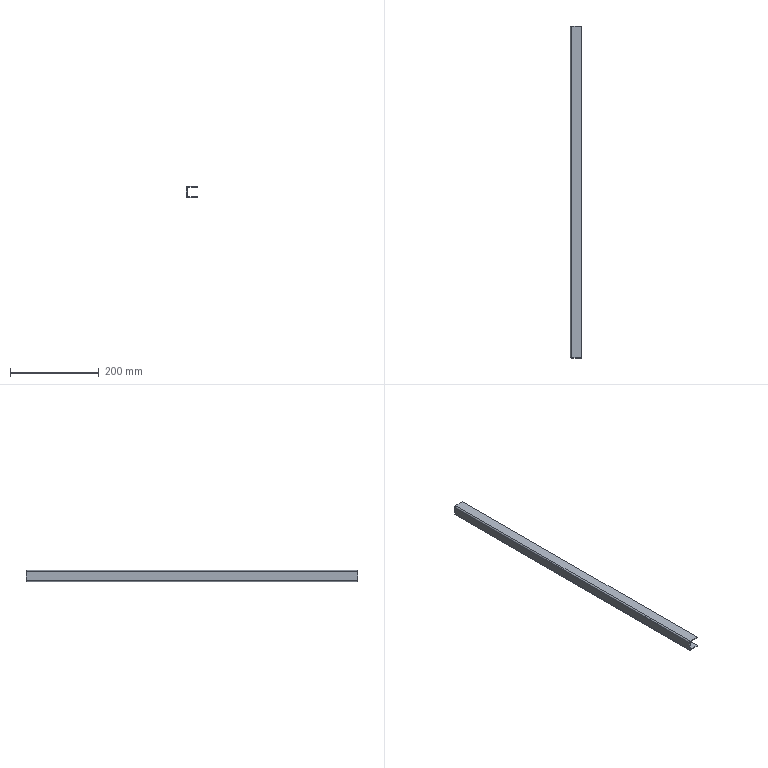Component | SolidWorks | Crossbeam.1(Item52)-1_Crossbeam.1(Item52)-1 | 1 solid | 22 faces | box 25 x 750 x 25 mm | volume 103925 mm3 | plane 18 | cylinder 4 | commonest cylinder face diameters 6 x2 2 x2 | material Plain Carbon Steel
STEP:
#1=CARTESIAN_POINT('',(-15.748,-14.764,-44.173));
#2=VERTEX_POINT('',#1);
#3=CARTESIAN_POINT('',(-15.669,-14.764,-44.173));
#4=VERTEX_POINT('',#3);
#5=CARTESIAN_POINT('',(-15.748,-14.764,-44.173));
#6=DIRECTION('',(1.,0.,-0.));
#7=VECTOR('',#6,39.37);
#8=LINE('',#5,#7);
#9=EDGE_CURVE('',#2,#4,#8,.T.);
#10=ORIENTED_EDGE('',*,*,#9,.F.);
#11=CARTESIAN_POINT('',(-15.63,-14.764,-44.291));
#12=VERTEX_POINT('',#11);
#13=CARTESIAN_POINT('',(-15.63,-14.764,-44.173));
#14=DIRECTION('',(-0.,1.,0.));
#15=DIRECTION('',(0.,0.,1.));
#16=AXIS2_PLACEMENT_3D('',#13,#14,#15);
#17=CIRCLE('',#16,0.1181);
#18=EDGE_CURVE('',#12,#2,#17,.T.);
#19=ORIENTED_EDGE('',*,*,#18,.F.);
#20=CARTESIAN_POINT('',(-15.63,-14.764,-44.213));
#21=VERTEX_POINT('',#20);
#22=CARTESIAN_POINT('',(-15.63,-14.764,-44.213));
#23=DIRECTION('',(-0.,0.,-1.));
#24=VECTOR('',#23,39.37);
#25=LINE('',#22,#24);
#26=EDGE_CURVE('',#21,#12,#25,.T.);
#27=ORIENTED_EDGE('',*,*,#26,.F.);
#28=CARTESIAN_POINT('',(-15.63,-14.764,-44.173));
#29=DIRECTION('',(-0.,1.,0.));
#30=DIRECTION('',(0.,0.,1.));
#31=AXIS2_PLACEMENT_3D('',#28,#29,#30);
#32=CIRCLE('',#31,0.03937);
#33=EDGE_CURVE('',#21,#4,#32,.T.);
#34=ORIENTED_EDGE('',*,*,#33,.T.);
#35=EDGE_LOOP('',(#10,#19,#27,#34));
#36=FACE_OUTER_BOUND('',#35,.T.);
#37=CARTESIAN_POINT('',(-15.748,-14.764,-44.173));
#38=DIRECTION('',(0.,-1.,-0.));
#39=DIRECTION('',(0.,-0.,1.));
#40=AXIS2_PLACEMENT_3D('',#37,#38,#39);
#41=PLANE('',#40);
#42=ADVANCED_FACE('',(#36),#41,.T.);
#43=CARTESIAN_POINT('',(-15.748,-14.764,-43.425));
#44=VERTEX_POINT('',#43);
#45=CARTESIAN_POINT('',(-15.748,-14.764,-44.291));
#46=DIRECTION('',(-0.,-0.,1.));
#47=VECTOR('',#46,39.37);
#48=LINE('',#45,#47);
#49=EDGE_CURVE('',#2,#44,#48,.T.);
#50=ORIENTED_EDGE('',*,*,#49,.F.);
#51=ORIENTED_EDGE('',*,*,#9,.T.);
#52=CARTESIAN_POINT('',(-15.669,-14.764,-43.425));
#53=VERTEX_POINT('',#52);
#54=CARTESIAN_POINT('',(-15.669,-14.764,-44.291));
#55=DIRECTION('',(-0.,-0.,1.));
#56=VECTOR('',#55,39.37);
#57=LINE('',#54,#56);
#58=EDGE_CURVE('',#4,#53,#57,.T.);
#59=ORIENTED_EDGE('',*,*,#58,.T.);
#60=CARTESIAN_POINT('',(-15.669,-14.764,-43.425));
#61=DIRECTION('',(-1.,-0.,0.));
#62=VECTOR('',#61,39.37);
#63=LINE('',#60,#62);
#64=EDGE_CURVE('',#53,#44,#63,.T.);
#65=ORIENTED_EDGE('',*,*,#64,.T.);
#66=EDGE_LOOP('',(#50,#51,#59,#65));
#67=FACE_OUTER_BOUND('',#66,.T.);
#68=CARTESIAN_POINT('',(-15.63,-14.764,-44.213));
#69=DIRECTION('',(0.,-1.,-0.));
#70=DIRECTION('',(0.,-0.,1.));
#71=AXIS2_PLACEMENT_3D('',#68,#69,#70);
#72=PLANE('',#71);
#73=ADVANCED_FACE('',(#67),#72,.T.);
#74=CARTESIAN_POINT('',(-15.63,14.764,-44.291));
#75=VERTEX_POINT('',#74);
#76=CARTESIAN_POINT('',(-15.63,14.764,-44.213));
#77=VERTEX_POINT('',#76);
#78=CARTESIAN_POINT('',(-15.63,14.764,-44.291));
#79=DIRECTION('',(0.,-0.,1.));
#80=VECTOR('',#79,39.37);
#81=LINE('',#78,#80);
#82=EDGE_CURVE('',#75,#77,#81,.T.);
#83=ORIENTED_EDGE('',*,*,#82,.F.);
#84=CARTESIAN_POINT('',(-15.748,14.764,-44.173));
#85=VERTEX_POINT('',#84);
#86=CARTESIAN_POINT('',(-15.63,14.764,-44.173));
#87=DIRECTION('',(-0.,1.,0.));
#88=DIRECTION('',(0.,0.,1.));
#89=AXIS2_PLACEMENT_3D('',#86,#87,#88);
#90=CIRCLE('',#89,0.1181);
#91=EDGE_CURVE('',#75,#85,#90,.T.);
#92=ORIENTED_EDGE('',*,*,#91,.T.);
#93=CARTESIAN_POINT('',(-15.669,14.764,-44.173));
#94=VERTEX_POINT('',#93);
#95=CARTESIAN_POINT('',(-15.669,14.764,-44.173));
#96=DIRECTION('',(-1.,-0.,0.));
#97=VECTOR('',#96,39.37);
#98=LINE('',#95,#97);
#99=EDGE_CURVE('',#94,#85,#98,.T.);
#100=ORIENTED_EDGE('',*,*,#99,.F.);
#101=CARTESIAN_POINT('',(-15.63,14.764,-44.173));
#102=DIRECTION('',(-0.,1.,0.));
#103=DIRECTION('',(0.,0.,1.));
#104=AXIS2_PLACEMENT_3D('',#101,#102,#103);
#105=CIRCLE('',#104,0.03937);
#106=EDGE_CURVE('',#77,#94,#105,.T.);
#107=ORIENTED_EDGE('',*,*,#106,.F.);
#108=EDGE_LOOP('',(#83,#92,#100,#107));
#109=FACE_OUTER_BOUND('',#108,.T.);
#110=CARTESIAN_POINT('',(-15.63,14.764,-44.291));
#111=DIRECTION('',(-0.,1.,0.));
#112=DIRECTION('',(-0.,0.,-1.));
#113=AXIS2_PLACEMENT_3D('',#110,#111,#112);
#114=PLANE('',#113);
#115=ADVANCED_FACE('',(#109),#114,.T.);
#116=CARTESIAN_POINT('',(-14.764,14.764,-44.291));
#117=VERTEX_POINT('',#116);
#118=CARTESIAN_POINT('',(-14.764,14.764,-44.291));
#119=DIRECTION('',(-1.,-0.,-0.));
#120=VECTOR('',#119,39.37);
#121=LINE('',#118,#120);
#122=EDGE_CURVE('',#117,#75,#121,.T.);
#123=ORIENTED_EDGE('',*,*,#122,.T.);
#124=ORIENTED_EDGE('',*,*,#82,.T.);
#125=CARTESIAN_POINT('',(-14.764,14.764,-44.213));
#126=VERTEX_POINT('',#125);
#127=CARTESIAN_POINT('',(-14.764,14.764,-44.213));
#128=DIRECTION('',(-1.,-0.,-0.));
#129=VECTOR('',#128,39.37);
#130=LINE('',#127,#129);
#131=EDGE_CURVE('',#126,#77,#130,.T.);
#132=ORIENTED_EDGE('',*,*,#131,.F.);
#133=CARTESIAN_POINT('',(-14.764,14.764,-44.213));
#134=DIRECTION('',(-0.,0.,-1.));
#135=VECTOR('',#134,39.37);
#136=LINE('',#133,#135);
#137=EDGE_CURVE('',#126,#117,#136,.T.);
#138=ORIENTED_EDGE('',*,*,#137,.T.);
#139=EDGE_LOOP('',(#123,#124,#132,#138));
#140=FACE_OUTER_BOUND('',#139,.T.);
#141=CARTESIAN_POINT('',(-15.669,14.764,-44.173));
#142=DIRECTION('',(-0.,1.,0.));
#143=DIRECTION('',(-0.,0.,-1.));
#144=AXIS2_PLACEMENT_3D('',#141,#142,#143);
#145=PLANE('',#144);
#146=ADVANCED_FACE('',(#140),#145,.T.);
#147=CARTESIAN_POINT('',(-15.63,-14.764,-43.307));
#148=VERTEX_POINT('',#147);
#149=CARTESIAN_POINT('',(-15.63,-14.764,-43.386));
#150=VERTEX_POINT('',#149);
#151=CARTESIAN_POINT('',(-15.63,-14.764,-43.307));
#152=DIRECTION('',(0.,0.,-1.));
#153=VECTOR('',#152,39.37);
#154=LINE('',#151,#153);
#155=EDGE_CURVE('',#148,#150,#154,.T.);
#156=ORIENTED_EDGE('',*,*,#155,.F.);
#157=CARTESIAN_POINT('',(-15.63,-14.764,-43.425));
#158=DIRECTION('',(-0.,1.,0.));
#159=DIRECTION('',(0.,0.,1.));
#160=AXIS2_PLACEMENT_3D('',#157,#158,#159);
#161=CIRCLE('',#160,0.1181);
#162=EDGE_CURVE('',#44,#148,#161,.T.);
#163=ORIENTED_EDGE('',*,*,#162,.F.);
#164=ORIENTED_EDGE('',*,*,#64,.F.);
#165=CARTESIAN_POINT('',(-15.63,-14.764,-43.425));
#166=DIRECTION('',(-0.,1.,0.));
#167=DIRECTION('',(0.,0.,1.));
#168=AXIS2_PLACEMENT_3D('',#165,#166,#167);
#169=CIRCLE('',#168,0.03937);
#170=EDGE_CURVE('',#53,#150,#169,.T.);
#171=ORIENTED_EDGE('',*,*,#170,.T.);
#172=EDGE_LOOP('',(#156,#163,#164,#171));
#173=FACE_OUTER_BOUND('',#172,.T.);
#174=CARTESIAN_POINT('',(-15.63,-14.764,-43.307));
#175=DIRECTION('',(0.,-1.,-0.));
#176=DIRECTION('',(0.,-0.,1.));
#177=AXIS2_PLACEMENT_3D('',#174,#175,#176);
#178=PLANE('',#177);
#179=ADVANCED_FACE('',(#173),#178,.T.);
#180=CARTESIAN_POINT('',(-14.764,-14.764,-43.307));
#181=VERTEX_POINT('',#180);
#182=CARTESIAN_POINT('',(-15.748,-14.764,-43.307));
#183=DIRECTION('',(1.,0.,0.));
#184=VECTOR('',#183,39.37);
#185=LINE('',#182,#184);
#186=EDGE_CURVE('',#148,#181,#185,.T.);
#187=ORIENTED_EDGE('',*,*,#186,.F.);
#188=ORIENTED_EDGE('',*,*,#155,.T.);
#189=CARTESIAN_POINT('',(-14.764,-14.764,-43.386));
#190=VERTEX_POINT('',#189);
#191=CARTESIAN_POINT('',(-15.748,-14.764,-43.386));
#192=DIRECTION('',(1.,0.,0.));
#193=VECTOR('',#192,39.37);
#194=LINE('',#191,#193);
#195=EDGE_CURVE('',#150,#190,#194,.T.);
#196=ORIENTED_EDGE('',*,*,#195,.T.);
#197=CARTESIAN_POINT('',(-14.764,-14.764,-43.307));
#198=DIRECTION('',(-0.,0.,-1.));
#199=VECTOR('',#198,39.37);
#200=LINE('',#197,#199);
#201=EDGE_CURVE('',#181,#190,#200,.T.);
#202=ORIENTED_EDGE('',*,*,#201,.F.);
#203=EDGE_LOOP('',(#187,#188,#196,#202));
#204=FACE_OUTER_BOUND('',#203,.T.);
#205=CARTESIAN_POINT('',(-15.669,-14.764,-43.425));
#206=DIRECTION('',(0.,-1.,-0.));
#207=DIRECTION('',(0.,-0.,1.));
#208=AXIS2_PLACEMENT_3D('',#205,#206,#207);
#209=PLANE('',#208);
#210=ADVANCED_FACE('',(#204),#209,.T.);
#211=CARTESIAN_POINT('',(-15.748,14.764,-43.425));
#212=VERTEX_POINT('',#211);
#213=CARTESIAN_POINT('',(-15.669,14.764,-43.425));
#214=VERTEX_POINT('',#213);
#215=CARTESIAN_POINT('',(-15.748,14.764,-43.425));
#216=DIRECTION('',(1.,0.,-0.));
#217=VECTOR('',#216,39.37);
#218=LINE('',#215,#217);
#219=EDGE_CURVE('',#212,#214,#218,.T.);
#220=ORIENTED_EDGE('',*,*,#219,.F.);
#221=CARTESIAN_POINT('',(-15.63,14.764,-43.307));
#222=VERTEX_POINT('',#221);
#223=CARTESIAN_POINT('',(-15.63,14.764,-43.425));
#224=DIRECTION('',(-0.,1.,0.));
#225=DIRECTION('',(0.,0.,1.));
#226=AXIS2_PLACEMENT_3D('',#223,#224,#225);
#227=CIRCLE('',#226,0.1181);
#228=EDGE_CURVE('',#212,#222,#227,.T.);
#229=ORIENTED_EDGE('',*,*,#228,.T.);
#230=CARTESIAN_POINT('',(-15.63,14.764,-43.386));
#231=VERTEX_POINT('',#230);
#232=CARTESIAN_POINT('',(-15.63,14.764,-43.386));
#233=DIRECTION('',(-0.,-0.,1.));
#234=VECTOR('',#233,39.37);
#235=LINE('',#232,#234);
#236=EDGE_CURVE('',#231,#222,#235,.T.);
#237=ORIENTED_EDGE('',*,*,#236,.F.);
#238=CARTESIAN_POINT('',(-15.63,14.764,-43.425));
#239=DIRECTION('',(-0.,1.,0.));
#240=DIRECTION('',(0.,0.,1.));
#241=AXIS2_PLACEMENT_3D('',#238,#239,#240);
#242=CIRCLE('',#241,0.03937);
#243=EDGE_CURVE('',#214,#231,#242,.T.);
#244=ORIENTED_EDGE('',*,*,#243,.F.);
#245=EDGE_LOOP('',(#220,#229,#237,#244));
#246=FACE_OUTER_BOUND('',#245,.T.);
#247=CARTESIAN_POINT('',(-15.748,14.764,-43.425));
#248=DIRECTION('',(-0.,1.,0.));
#249=DIRECTION('',(-0.,0.,-1.));
#250=AXIS2_PLACEMENT_3D('',#247,#248,#249);
#251=PLANE('',#250);
#252=ADVANCED_FACE('',(#246),#251,.T.);
#253=CARTESIAN_POINT('',(-15.748,14.764,-44.291));
#254=DIRECTION('',(-0.,-0.,1.));
#255=VECTOR('',#254,39.37);
#256=LINE('',#253,#255);
#257=EDGE_CURVE('',#85,#212,#256,.T.);
#258=ORIENTED_EDGE('',*,*,#257,.T.);
#259=ORIENTED_EDGE('',*,*,#219,.T.);
#260=CARTESIAN_POINT('',(-15.669,14.764,-44.291));
#261=DIRECTION('',(-0.,-0.,1.));
#262=VECTOR('',#261,39.37);
#263=LINE('',#260,#262);
#264=EDGE_CURVE('',#94,#214,#263,.T.);
#265=ORIENTED_EDGE('',*,*,#264,.F.);
#266=ORIENTED_EDGE('',*,*,#99,.T.);
#267=EDGE_LOOP('',(#258,#259,#265,#266));
#268=FACE_OUTER_BOUND('',#267,.T.);
#269=CARTESIAN_POINT('',(-15.63,14.764,-43.386));
#270=DIRECTION('',(-0.,1.,0.));
#271=DIRECTION('',(-0.,0.,-1.));
#272=AXIS2_PLACEMENT_3D('',#269,#270,#271);
#273=PLANE('',#272);
#274=ADVANCED_FACE('',(#268),#273,.T.);
#275=CARTESIAN_POINT('',(-14.764,14.764,-43.386));
#276=VERTEX_POINT('',#275);
#277=CARTESIAN_POINT('',(-15.748,14.764,-43.386));
#278=DIRECTION('',(1.,0.,0.));
#279=VECTOR('',#278,39.37);
#280=LINE('',#277,#279);
#281=EDGE_CURVE('',#231,#276,#280,.T.);
#282=ORIENTED_EDGE('',*,*,#281,.T.);
#283=CARTESIAN_POINT('',(-14.764,-14.764,-43.386));
#284=DIRECTION('',(-0.,1.,0.));
#285=VECTOR('',#284,39.37);
#286=LINE('',#283,#285);
#287=EDGE_CURVE('',#190,#276,#286,.T.);
#288=ORIENTED_EDGE('',*,*,#287,.F.);
#289=ORIENTED_EDGE('',*,*,#195,.F.);
#290=CARTESIAN_POINT('',(-15.63,-14.764,-43.386));
#291=DIRECTION('',(-0.,1.,0.));
#292=VECTOR('',#291,39.37);
#293=LINE('',#290,#292);
#294=EDGE_CURVE('',#150,#231,#293,.T.);
#295=ORIENTED_EDGE('',*,*,#294,.T.);
#296=EDGE_LOOP('',(#282,#288,#289,#295));
#297=FACE_OUTER_BOUND('',#296,.T.);
#298=CARTESIAN_POINT('',(-15.748,-14.764,-43.386));
#299=DIRECTION('',(-0.,-0.,1.));
#300=DIRECTION('',(-1.,-0.,-0.));
#301=AXIS2_PLACEMENT_3D('',#298,#299,#300);
#302=PLANE('',#301);
#303=ADVANCED_FACE('',(#297),#302,.F.);
#304=CARTESIAN_POINT('',(-14.764,14.764,-43.307));
#305=VERTEX_POINT('',#304);
#306=CARTESIAN_POINT('',(-14.764,14.764,-43.307));
#307=DIRECTION('',(-0.,0.,-1.));
#308=VECTOR('',#307,39.37);
#309=LINE('',#306,#308);
#310=EDGE_CURVE('',#305,#276,#309,.T.);
#311=ORIENTED_EDGE('',*,*,#310,.F.);
#312=CARTESIAN_POINT('',(-14.764,-14.764,-43.307));
#313=DIRECTION('',(-0.,1.,0.));
#314=VECTOR('',#313,39.37);
#315=LINE('',#312,#314);
#316=EDGE_CURVE('',#181,#305,#315,.T.);
#317=ORIENTED_EDGE('',*,*,#316,.F.);
#318=ORIENTED_EDGE('',*,*,#201,.T.);
#319=ORIENTED_EDGE('',*,*,#287,.T.);
#320=EDGE_LOOP('',(#311,#317,#318,#319));
#321=FACE_OUTER_BOUND('',#320,.T.);
#322=CARTESIAN_POINT('',(-14.764,-14.764,-43.307));
#323=DIRECTION('',(1.,0.,-0.));
#324=DIRECTION('',(-0.,1.,0.));
#325=AXIS2_PLACEMENT_3D('',#322,#323,#324);
#326=PLANE('',#325);
#327=ADVANCED_FACE('',(#321),#326,.T.);
#328=CARTESIAN_POINT('',(-15.748,14.764,-43.307));
#329=DIRECTION('',(1.,0.,0.));
#330=VECTOR('',#329,39.37);
#331=LINE('',#328,#330);
#332=EDGE_CURVE('',#222,#305,#331,.T.);
#333=ORIENTED_EDGE('',*,*,#332,.F.);
#334=CARTESIAN_POINT('',(-15.63,-14.764,-43.307));
#335=DIRECTION('',(-0.,1.,0.));
#336=VECTOR('',#335,39.37);
#337=LINE('',#334,#336);
#338=EDGE_CURVE('',#148,#222,#337,.T.);
#339=ORIENTED_EDGE('',*,*,#338,.F.);
#340=ORIENTED_EDGE('',*,*,#186,.T.);
#341=ORIENTED_EDGE('',*,*,#316,.T.);
#342=EDGE_LOOP('',(#333,#339,#340,#341));
#343=FACE_OUTER_BOUND('',#342,.T.);
#344=CARTESIAN_POINT('',(-15.748,-14.764,-43.307));
#345=DIRECTION('',(-0.,-0.,1.));
#346=DIRECTION('',(-1.,-0.,-0.));
#347=AXIS2_PLACEMENT_3D('',#344,#345,#346);
#348=PLANE('',#347);
#349=ADVANCED_FACE('',(#343),#348,.T.);
#350=ORIENTED_EDGE('',*,*,#228,.F.);
#351=CARTESIAN_POINT('',(-15.748,-14.764,-43.425));
#352=DIRECTION('',(-0.,1.,0.));
#353=VECTOR('',#352,39.37);
#354=LINE('',#351,#353);
#355=EDGE_CURVE('',#44,#212,#354,.T.);
#356=ORIENTED_EDGE('',*,*,#355,.F.);
#357=ORIENTED_EDGE('',*,*,#162,.T.);
#358=ORIENTED_EDGE('',*,*,#338,.T.);
#359=EDGE_LOOP('',(#350,#356,#357,#358));
#360=FACE_OUTER_BOUND('',#359,.T.);
#361=CARTESIAN_POINT('',(-15.63,-14.764,-43.425));
#362=DIRECTION('',(-0.,1.,0.));
#363=DIRECTION('',(0.,0.,-1.));
#364=AXIS2_PLACEMENT_3D('',#361,#362,#363);
#365=CYLINDRICAL_SURFACE('',#364,0.1181);
#366=ADVANCED_FACE('',(#360),#365,.T.);
#367=ORIENTED_EDGE('',*,*,#257,.F.);
#368=CARTESIAN_POINT('',(-15.748,-14.764,-44.173));
#369=DIRECTION('',(-0.,1.,0.));
#370=VECTOR('',#369,39.37);
#371=LINE('',#368,#370);
#372=EDGE_CURVE('',#2,#85,#371,.T.);
#373=ORIENTED_EDGE('',*,*,#372,.F.);
#374=ORIENTED_EDGE('',*,*,#49,.T.);
#375=ORIENTED_EDGE('',*,*,#355,.T.);
#376=EDGE_LOOP('',(#367,#373,#374,#375));
#377=FACE_OUTER_BOUND('',#376,.T.);
#378=CARTESIAN_POINT('',(-15.748,-14.764,-44.291));
#379=DIRECTION('',(-1.,-0.,-0.));
#380=DIRECTION('',(0.,0.,-1.));
#381=AXIS2_PLACEMENT_3D('',#378,#379,#380);
#382=PLANE('',#381);
#383=ADVANCED_FACE('',(#377),#382,.T.);
#384=ORIENTED_EDGE('',*,*,#91,.F.);
#385=CARTESIAN_POINT('',(-15.63,-14.764,-44.291));
#386=DIRECTION('',(-0.,1.,0.));
#387=VECTOR('',#386,39.37);
#388=LINE('',#385,#387);
#389=EDGE_CURVE('',#12,#75,#388,.T.);
#390=ORIENTED_EDGE('',*,*,#389,.F.);
#391=ORIENTED_EDGE('',*,*,#18,.T.);
#392=ORIENTED_EDGE('',*,*,#372,.T.);
#393=EDGE_LOOP('',(#384,#390,#391,#392));
#394=FACE_OUTER_BOUND('',#393,.T.);
#395=CARTESIAN_POINT('',(-15.63,-14.764,-44.173));
#396=DIRECTION('',(-0.,1.,0.));
#397=DIRECTION('',(0.,0.,-1.));
#398=AXIS2_PLACEMENT_3D('',#395,#396,#397);
#399=CYLINDRICAL_SURFACE('',#398,0.1181);
#400=ADVANCED_FACE('',(#394),#399,.T.);
#401=ORIENTED_EDGE('',*,*,#122,.F.);
#402=CARTESIAN_POINT('',(-14.764,-14.764,-44.291));
#403=VERTEX_POINT('',#402);
#404=CARTESIAN_POINT('',(-14.764,-14.764,-44.291));
#405=DIRECTION('',(-0.,1.,0.));
#406=VECTOR('',#405,39.37);
#407=LINE('',#404,#406);
#408=EDGE_CURVE('',#403,#117,#407,.T.);
#409=ORIENTED_EDGE('',*,*,#408,.F.);
#410=CARTESIAN_POINT('',(-14.764,-14.764,-44.291));
#411=DIRECTION('',(-1.,-0.,-0.));
#412=VECTOR('',#411,39.37);
#413=LINE('',#410,#412);
#414=EDGE_CURVE('',#403,#12,#413,.T.);
#415=ORIENTED_EDGE('',*,*,#414,.T.);
#416=ORIENTED_EDGE('',*,*,#389,.T.);
#417=EDGE_LOOP('',(#401,#409,#415,#416));
#418=FACE_OUTER_BOUND('',#417,.T.);
#419=CARTESIAN_POINT('',(-14.764,-14.764,-44.291));
#420=DIRECTION('',(0.,0.,-1.));
#421=DIRECTION('',(1.,0.,0.));
#422=AXIS2_PLACEMENT_3D('',#419,#420,#421);
#423=PLANE('',#422);
#424=ADVANCED_FACE('',(#418),#423,.T.);
#425=ORIENTED_EDGE('',*,*,#137,.F.);
#426=CARTESIAN_POINT('',(-14.764,-14.764,-44.213));
#427=VERTEX_POINT('',#426);
#428=CARTESIAN_POINT('',(-14.764,-14.764,-44.213));
#429=DIRECTION('',(-0.,1.,0.));
#430=VECTOR('',#429,39.37);
#431=LINE('',#428,#430);
#432=EDGE_CURVE('',#427,#126,#431,.T.);
#433=ORIENTED_EDGE('',*,*,#432,.F.);
#434=CARTESIAN_POINT('',(-14.764,-14.764,-44.213));
#435=DIRECTION('',(-0.,0.,-1.));
#436=VECTOR('',#435,39.37);
#437=LINE('',#434,#436);
#438=EDGE_CURVE('',#427,#403,#437,.T.);
#439=ORIENTED_EDGE('',*,*,#438,.T.);
#440=ORIENTED_EDGE('',*,*,#408,.T.);
#441=EDGE_LOOP('',(#425,#433,#439,#440));
#442=FACE_OUTER_BOUND('',#441,.T.);
#443=CARTESIAN_POINT('',(-14.764,-14.764,-44.213));
#444=DIRECTION('',(1.,0.,-0.));
#445=DIRECTION('',(-0.,1.,0.));
#446=AXIS2_PLACEMENT_3D('',#443,#444,#445);
#447=PLANE('',#446);
#448=ADVANCED_FACE('',(#442),#447,.T.);
#449=ORIENTED_EDGE('',*,*,#131,.T.);
#450=CARTESIAN_POINT('',(-15.63,-14.764,-44.213));
#451=DIRECTION('',(-0.,1.,0.));
#452=VECTOR('',#451,39.37);
#453=LINE('',#450,#452);
#454=EDGE_CURVE('',#21,#77,#453,.T.);
#455=ORIENTED_EDGE('',*,*,#454,.F.);
#456=CARTESIAN_POINT('',(-14.764,-14.764,-44.213));
#457=DIRECTION('',(-1.,-0.,-0.));
#458=VECTOR('',#457,39.37);
#459=LINE('',#456,#458);
#460=EDGE_CURVE('',#427,#21,#459,.T.);
#461=ORIENTED_EDGE('',*,*,#460,.F.);
#462=ORIENTED_EDGE('',*,*,#432,.T.);
#463=EDGE_LOOP('',(#449,#455,#461,#462));
#464=FACE_OUTER_BOUND('',#463,.T.);
#465=CARTESIAN_POINT('',(-14.764,-14.764,-44.213));
#466=DIRECTION('',(0.,0.,-1.));
#467=DIRECTION('',(1.,0.,0.));
#468=AXIS2_PLACEMENT_3D('',#465,#466,#467);
#469=PLANE('',#468);
#470=ADVANCED_FACE('',(#464),#469,.F.);
#471=ORIENTED_EDGE('',*,*,#106,.T.);
#472=CARTESIAN_POINT('',(-15.669,-14.764,-44.173));
#473=DIRECTION('',(-0.,1.,0.));
#474=VECTOR('',#473,39.37);
#475=LINE('',#472,#474);
#476=EDGE_CURVE('',#4,#94,#475,.T.);
#477=ORIENTED_EDGE('',*,*,#476,.F.);
#478=ORIENTED_EDGE('',*,*,#33,.F.);
#479=ORIENTED_EDGE('',*,*,#454,.T.);
#480=EDGE_LOOP('',(#471,#477,#478,#479));
#481=FACE_OUTER_BOUND('',#480,.T.);
#482=CARTESIAN_POINT('',(-15.63,-14.764,-44.173));
#483=DIRECTION('',(-0.,1.,0.));
#484=DIRECTION('',(0.,0.,-1.));
#485=AXIS2_PLACEMENT_3D('',#482,#483,#484);
#486=CYLINDRICAL_SURFACE('',#485,0.03937);
#487=ADVANCED_FACE('',(#481),#486,.F.);
#488=ORIENTED_EDGE('',*,*,#264,.T.);
#489=CARTESIAN_POINT('',(-15.669,-14.764,-43.425));
#490=DIRECTION('',(-0.,1.,0.));
#491=VECTOR('',#490,39.37);
#492=LINE('',#489,#491);
#493=EDGE_CURVE('',#53,#214,#492,.T.);
#494=ORIENTED_EDGE('',*,*,#493,.F.);
#495=ORIENTED_EDGE('',*,*,#58,.F.);
#496=ORIENTED_EDGE('',*,*,#476,.T.);
#497=EDGE_LOOP('',(#488,#494,#495,#496));
#498=FACE_OUTER_BOUND('',#497,.T.);
#499=CARTESIAN_POINT('',(-15.669,-14.764,-44.291));
#500=DIRECTION('',(-1.,-0.,-0.));
#501=DIRECTION('',(0.,0.,-1.));
#502=AXIS2_PLACEMENT_3D('',#499,#500,#501);
#503=PLANE('',#502);
#504=ADVANCED_FACE('',(#498),#503,.F.);
#505=ORIENTED_EDGE('',*,*,#243,.T.);
#506=ORIENTED_EDGE('',*,*,#294,.F.);
#507=ORIENTED_EDGE('',*,*,#170,.F.);
#508=ORIENTED_EDGE('',*,*,#493,.T.);
#509=EDGE_LOOP('',(#505,#506,#507,#508));
#510=FACE_OUTER_BOUND('',#509,.T.);
#511=CARTESIAN_POINT('',(-15.63,-14.764,-43.425));
#512=DIRECTION('',(-0.,1.,0.));
#513=DIRECTION('',(0.,0.,-1.));
#514=AXIS2_PLACEMENT_3D('',#511,#512,#513);
#515=CYLINDRICAL_SURFACE('',#514,0.03937);
#516=ADVANCED_FACE('',(#510),#515,.F.);
#517=ORIENTED_EDGE('',*,*,#460,.T.);
#518=ORIENTED_EDGE('',*,*,#26,.T.);
#519=ORIENTED_EDGE('',*,*,#414,.F.);
#520=ORIENTED_EDGE('',*,*,#438,.F.);
#521=EDGE_LOOP('',(#517,#518,#519,#520));
#522=FACE_OUTER_BOUND('',#521,.T.);
#523=CARTESIAN_POINT('',(-15.63,-14.764,-43.425));
#524=DIRECTION('',(0.,-1.,-0.));
#525=DIRECTION('',(0.,-0.,1.));
#526=AXIS2_PLACEMENT_3D('',#523,#524,#525);
#527=PLANE('',#526);
#528=ADVANCED_FACE('',(#522),#527,.T.);
#529=ORIENTED_EDGE('',*,*,#281,.F.);
#530=ORIENTED_EDGE('',*,*,#236,.T.);
#531=ORIENTED_EDGE('',*,*,#332,.T.);
#532=ORIENTED_EDGE('',*,*,#310,.T.);
#533=EDGE_LOOP('',(#529,#530,#531,#532));
#534=FACE_OUTER_BOUND('',#533,.T.);
#535=CARTESIAN_POINT('',(-15.63,14.764,-43.425));
#536=DIRECTION('',(0.,-1.,-0.));
#537=DIRECTION('',(0.,-0.,1.));
#538=AXIS2_PLACEMENT_3D('',#535,#536,#537);
#539=PLANE('',#538);
#540=ADVANCED_FACE('',(#534),#539,.F.);
#541=CLOSED_SHELL('',(#42,#73,#115,#146,#179,#210,#252,#274,#303,#327,#349,#366,#383,#400,#424,#448,#470,#487,#504,#516,#528,#540));
#542=MANIFOLD_SOLID_BREP('',#541);
#543=CARTESIAN_POINT('',(0.,0.,0.));
#544=DIRECTION('',(0.,0.,1.));
#545=DIRECTION('',(1.,0.,0.));
#546=AXIS2_PLACEMENT_3D('',#543,#544,#545);
#547=(LENGTH_UNIT()NAMED_UNIT(*)SI_UNIT($,.METRE.));
#548=LENGTH_MEASURE_WITH_UNIT(LENGTH_MEASURE(0.0254),#547);
#549=DIMENSIONAL_EXPONENTS(1.,0.,0.,0.,0.,0.,0.);
#550=(CONVERSION_BASED_UNIT('',#548)LENGTH_UNIT()NAMED_UNIT(#549));
#551=UNCERTAINTY_MEASURE_WITH_UNIT(LENGTH_MEASURE(0.00001),#550,'','');
#552=(NAMED_UNIT(*)PLANE_ANGLE_UNIT()SI_UNIT($,.RADIAN.));
#553=(NAMED_UNIT(*)SI_UNIT($,.STERADIAN.)SOLID_ANGLE_UNIT());
#554=(GEOMETRIC_REPRESENTATION_CONTEXT(3)GLOBAL_UNCERTAINTY_ASSIGNED_CONTEXT((#551))GLOBAL_UNIT_ASSIGNED_CONTEXT((#550,#552,#553))REPRESENTATION_CONTEXT('',''));
#555=ADVANCED_BREP_SHAPE_REPRESENTATION('',(#542,#546),#554);
#556=COLOUR_RGB('',0.7922,0.8196,0.9333);
#557=FILL_AREA_STYLE_COLOUR('',#556);
#558=FILL_AREA_STYLE('',(#557));
#559=SURFACE_STYLE_FILL_AREA(#558);
#560=SURFACE_SIDE_STYLE('',(#559));
#561=SURFACE_STYLE_USAGE(.BOTH.,#560);
#562=PRESENTATION_STYLE_ASSIGNMENT((#561));
#563=STYLED_ITEM('',(#562),#542);
#564=(LENGTH_UNIT()NAMED_UNIT(*)SI_UNIT($,.METRE.));
#565=LENGTH_MEASURE_WITH_UNIT(LENGTH_MEASURE(0.0254),#564);
#566=DIMENSIONAL_EXPONENTS(1.,0.,0.,0.,0.,0.,0.);
#567=(CONVERSION_BASED_UNIT('',#565)LENGTH_UNIT()NAMED_UNIT(#566));
#568=UNCERTAINTY_MEASURE_WITH_UNIT(LENGTH_MEASURE(0.00001),#567,'','');
#569=(NAMED_UNIT(*)PLANE_ANGLE_UNIT()SI_UNIT($,.RADIAN.));
#570=(NAMED_UNIT(*)SI_UNIT($,.STERADIAN.)SOLID_ANGLE_UNIT());
#571=(GEOMETRIC_REPRESENTATION_CONTEXT(3)GLOBAL_UNCERTAINTY_ASSIGNED_CONTEXT((#568))GLOBAL_UNIT_ASSIGNED_CONTEXT((#567,#569,#570))REPRESENTATION_CONTEXT('',''));
#572=MECHANICAL_DESIGN_GEOMETRIC_PRESENTATION_REPRESENTATION('',(#563),#571);
#573=PRESENTATION_LAYER_ASSIGNMENT('','',(#563));